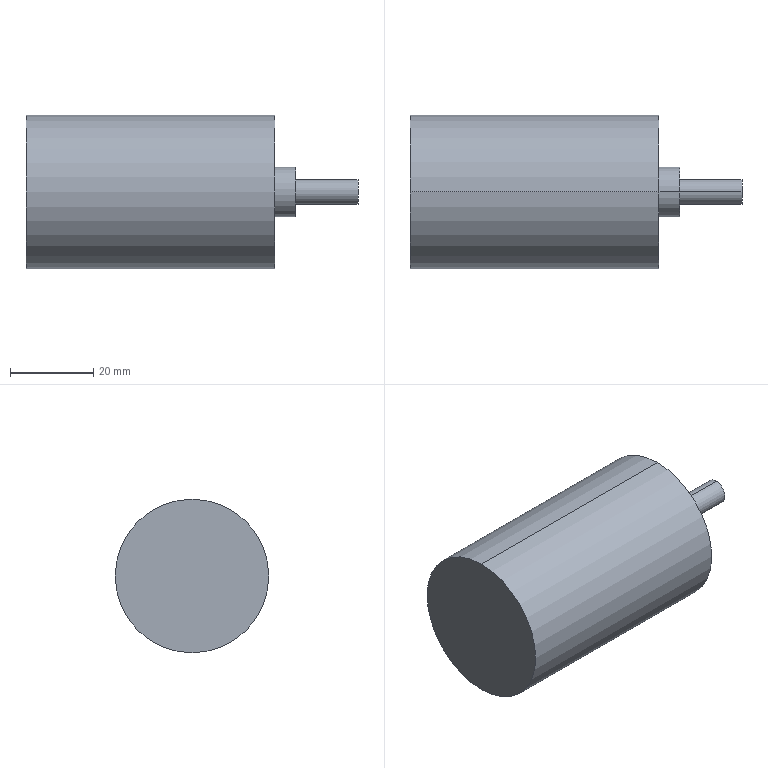Component | SolidWorks | AS-011-JG0105-1 | 1 solid | 34 faces | box 80 x 37 x 37 mm | volume 65244 mm3 | cylinder 18 | cone 12 | plane 4 | commonest cylinder face diameters 2.5 x12 6 x2 12 x2 37 x2
build123d program:
from build123d import *

# Parameters (mm, degrees)
M3_TAPPED_HOLE1_D     = 2.5
M3_TAPPED_HOLE1_DEPTH = 8.5
M3_TAPPED_HOLE1_TIP   = 0.7511


with BuildPart() as part:
    # Sketch1 → Revolve1 (revolve)
    with BuildSketch(Plane.XY, mode=Mode.PRIVATE) as revolve1_sk:
        Polygon((80, 3), (65, 3), (65, 6), (60, 6), (60, 18.5), (0, 18.5), (0, 0), (80, 0), align=None)
    revolve(revolve1_sk.sketch.rotate(Axis((80, 0, 0), (-1, 0, 0)), 90), axis=Axis((80, 0, 0), (-1, 0, 0)))

    # M3 Tapped Hole1
    with Locations(Plane(origin=(60, 0, 0), x_dir=(0, 0, -1), z_dir=(1, 0, 0))):
        with Locations((7.75, 13.423), (-7.75, 13.423), (15.5, 0), (-15.5, 0), (-7.75, -13.423), (7.75, -13.423)):
            Hole(M3_TAPPED_HOLE1_D / 2, depth=M3_TAPPED_HOLE1_DEPTH)
            with Locations((0, 0, -(M3_TAPPED_HOLE1_DEPTH + M3_TAPPED_HOLE1_TIP / 2))):  # 118° drill point
                Cone(0, M3_TAPPED_HOLE1_D / 2, M3_TAPPED_HOLE1_TIP, mode=Mode.SUBTRACT)


solid = part.part

# Placed as in the assembly
solid = solid.moved(Location((-97, -18, -10), (0, 0, 0)))
STEP:
#1=CARTESIAN_POINT('',(-1.791,-0.1802,-0.6496));
#2=VERTEX_POINT('',#1);
#3=CARTESIAN_POINT('',(-1.791,-0.1802,-0.748));
#4=VERTEX_POINT('',#3);
#5=CARTESIAN_POINT('',(-1.791,-0.1802,-0.6988));
#6=DIRECTION('',(1.,0.,0.));
#7=DIRECTION('',(0.,0.,-1.));
#8=AXIS2_PLACEMENT_3D('',#5,#6,#7);
#9=CIRCLE('',#8,0.04921);
#10=EDGE_CURVE('',#2,#4,#9,.T.);
#11=ORIENTED_EDGE('',*,*,#10,.F.);
#12=CARTESIAN_POINT('',(-1.457,-0.1802,-0.6496));
#13=VERTEX_POINT('',#12);
#14=CARTESIAN_POINT('',(-1.457,-0.1802,-0.6496));
#15=DIRECTION('',(1.,0.,0.));
#16=VECTOR('',#15,39.37);
#17=LINE('',#14,#16);
#18=EDGE_CURVE('',#2,#13,#17,.T.);
#19=ORIENTED_EDGE('',*,*,#18,.T.);
#20=CARTESIAN_POINT('',(-1.457,-0.1802,-0.748));
#21=VERTEX_POINT('',#20);
#22=CARTESIAN_POINT('',(-1.457,-0.1802,-0.6988));
#23=DIRECTION('',(1.,0.,0.));
#24=DIRECTION('',(0.,0.,-1.));
#25=AXIS2_PLACEMENT_3D('',#22,#23,#24);
#26=CIRCLE('',#25,0.04921);
#27=EDGE_CURVE('',#13,#21,#26,.T.);
#28=ORIENTED_EDGE('',*,*,#27,.T.);
#29=CARTESIAN_POINT('',(-1.457,-0.1802,-0.748));
#30=DIRECTION('',(1.,0.,0.));
#31=VECTOR('',#30,39.37);
#32=LINE('',#29,#31);
#33=EDGE_CURVE('',#4,#21,#32,.T.);
#34=ORIENTED_EDGE('',*,*,#33,.F.);
#35=EDGE_LOOP('',(#11,#19,#28,#34));
#36=FACE_OUTER_BOUND('',#35,.T.);
#37=CARTESIAN_POINT('',(-1.457,-0.1802,-0.6988));
#38=DIRECTION('',(1.,0.,0.));
#39=DIRECTION('',(0.,0.,-1.));
#40=AXIS2_PLACEMENT_3D('',#37,#38,#39);
#41=CYLINDRICAL_SURFACE('',#40,0.04921);
#42=ADVANCED_FACE('',(#36),#41,.F.);
#43=CARTESIAN_POINT('',(-1.821,-0.1802,-0.6988));
#44=VERTEX_POINT('',#43);
#45=CARTESIAN_POINT('',(-1.791,-0.1802,-0.748));
#46=DIRECTION('',(0.515,0.,-0.8572));
#47=VECTOR('',#46,39.37);
#48=LINE('',#45,#47);
#49=EDGE_CURVE('',#44,#4,#48,.T.);
#50=ORIENTED_EDGE('',*,*,#49,.F.);
#51=CARTESIAN_POINT('',(-1.791,-0.1802,-0.6496));
#52=DIRECTION('',(0.515,0.,0.8572));
#53=VECTOR('',#52,39.37);
#54=LINE('',#51,#53);
#55=EDGE_CURVE('',#44,#2,#54,.T.);
#56=ORIENTED_EDGE('',*,*,#55,.T.);
#57=ORIENTED_EDGE('',*,*,#10,.T.);
#58=EDGE_LOOP('',(#50,#56,#57));
#59=FACE_OUTER_BOUND('',#58,.T.);
#60=CARTESIAN_POINT('',(-1.791,-0.1802,-0.6988));
#61=DIRECTION('',(1.,0.,0.));
#62=DIRECTION('',(0.,0.,-1.));
#63=AXIS2_PLACEMENT_3D('',#60,#61,#62);
#64=CONICAL_SURFACE('',#63,0.04921,1.03);
#65=ADVANCED_FACE('',(#59),#64,.F.);
#66=CARTESIAN_POINT('',(-1.791,-0.1802,-0.03937));
#67=VERTEX_POINT('',#66);
#68=CARTESIAN_POINT('',(-1.791,-0.1802,-0.1378));
#69=VERTEX_POINT('',#68);
#70=CARTESIAN_POINT('',(-1.791,-0.1802,-0.08858));
#71=DIRECTION('',(1.,0.,0.));
#72=DIRECTION('',(0.,0.,-1.));
#73=AXIS2_PLACEMENT_3D('',#70,#71,#72);
#74=CIRCLE('',#73,0.04921);
#75=EDGE_CURVE('',#67,#69,#74,.T.);
#76=ORIENTED_EDGE('',*,*,#75,.F.);
#77=CARTESIAN_POINT('',(-1.457,-0.1802,-0.03937));
#78=VERTEX_POINT('',#77);
#79=CARTESIAN_POINT('',(-1.457,-0.1802,-0.03937));
#80=DIRECTION('',(1.,0.,0.));
#81=VECTOR('',#80,39.37);
#82=LINE('',#79,#81);
#83=EDGE_CURVE('',#67,#78,#82,.T.);
#84=ORIENTED_EDGE('',*,*,#83,.T.);
#85=CARTESIAN_POINT('',(-1.457,-0.1802,-0.1378));
#86=VERTEX_POINT('',#85);
#87=CARTESIAN_POINT('',(-1.457,-0.1802,-0.08858));
#88=DIRECTION('',(1.,0.,0.));
#89=DIRECTION('',(0.,0.,-1.));
#90=AXIS2_PLACEMENT_3D('',#87,#88,#89);
#91=CIRCLE('',#90,0.04921);
#92=EDGE_CURVE('',#78,#86,#91,.T.);
#93=ORIENTED_EDGE('',*,*,#92,.T.);
#94=CARTESIAN_POINT('',(-1.457,-0.1802,-0.1378));
#95=DIRECTION('',(1.,0.,0.));
#96=VECTOR('',#95,39.37);
#97=LINE('',#94,#96);
#98=EDGE_CURVE('',#69,#86,#97,.T.);
#99=ORIENTED_EDGE('',*,*,#98,.F.);
#100=EDGE_LOOP('',(#76,#84,#93,#99));
#101=FACE_OUTER_BOUND('',#100,.T.);
#102=CARTESIAN_POINT('',(-1.457,-0.1802,-0.08858));
#103=DIRECTION('',(1.,0.,0.));
#104=DIRECTION('',(0.,0.,-1.));
#105=AXIS2_PLACEMENT_3D('',#102,#103,#104);
#106=CYLINDRICAL_SURFACE('',#105,0.04921);
#107=ADVANCED_FACE('',(#101),#106,.F.);
#108=CARTESIAN_POINT('',(-1.821,-0.1802,-0.08858));
#109=VERTEX_POINT('',#108);
#110=CARTESIAN_POINT('',(-1.791,-0.1802,-0.1378));
#111=DIRECTION('',(0.515,0.,-0.8572));
#112=VECTOR('',#111,39.37);
#113=LINE('',#110,#112);
#114=EDGE_CURVE('',#109,#69,#113,.T.);
#115=ORIENTED_EDGE('',*,*,#114,.F.);
#116=CARTESIAN_POINT('',(-1.791,-0.1802,-0.03937));
#117=DIRECTION('',(0.515,0.,0.8572));
#118=VECTOR('',#117,39.37);
#119=LINE('',#116,#118);
#120=EDGE_CURVE('',#109,#67,#119,.T.);
#121=ORIENTED_EDGE('',*,*,#120,.T.);
#122=ORIENTED_EDGE('',*,*,#75,.T.);
#123=EDGE_LOOP('',(#115,#121,#122));
#124=FACE_OUTER_BOUND('',#123,.T.);
#125=CARTESIAN_POINT('',(-1.791,-0.1802,-0.08858));
#126=DIRECTION('',(1.,0.,0.));
#127=DIRECTION('',(0.,0.,-1.));
#128=AXIS2_PLACEMENT_3D('',#125,#126,#127);
#129=CONICAL_SURFACE('',#128,0.04921,1.03);
#130=ADVANCED_FACE('',(#124),#129,.F.);
#131=CARTESIAN_POINT('',(-1.791,-0.7087,-0.9547));
#132=VERTEX_POINT('',#131);
#133=CARTESIAN_POINT('',(-1.791,-0.7087,-1.053));
#134=VERTEX_POINT('',#133);
#135=CARTESIAN_POINT('',(-1.791,-0.7087,-1.004));
#136=DIRECTION('',(1.,0.,0.));
#137=DIRECTION('',(0.,0.,-1.));
#138=AXIS2_PLACEMENT_3D('',#135,#136,#137);
#139=CIRCLE('',#138,0.04921);
#140=EDGE_CURVE('',#132,#134,#139,.T.);
#141=ORIENTED_EDGE('',*,*,#140,.F.);
#142=CARTESIAN_POINT('',(-1.457,-0.7087,-0.9547));
#143=VERTEX_POINT('',#142);
#144=CARTESIAN_POINT('',(-1.457,-0.7087,-0.9547));
#145=DIRECTION('',(1.,0.,0.));
#146=VECTOR('',#145,39.37);
#147=LINE('',#144,#146);
#148=EDGE_CURVE('',#132,#143,#147,.T.);
#149=ORIENTED_EDGE('',*,*,#148,.T.);
#150=CARTESIAN_POINT('',(-1.457,-0.7087,-1.053));
#151=VERTEX_POINT('',#150);
#152=CARTESIAN_POINT('',(-1.457,-0.7087,-1.004));
#153=DIRECTION('',(1.,0.,0.));
#154=DIRECTION('',(0.,0.,-1.));
#155=AXIS2_PLACEMENT_3D('',#152,#153,#154);
#156=CIRCLE('',#155,0.04921);
#157=EDGE_CURVE('',#143,#151,#156,.T.);
#158=ORIENTED_EDGE('',*,*,#157,.T.);
#159=CARTESIAN_POINT('',(-1.457,-0.7087,-1.053));
#160=DIRECTION('',(1.,0.,0.));
#161=VECTOR('',#160,39.37);
#162=LINE('',#159,#161);
#163=EDGE_CURVE('',#134,#151,#162,.T.);
#164=ORIENTED_EDGE('',*,*,#163,.F.);
#165=EDGE_LOOP('',(#141,#149,#158,#164));
#166=FACE_OUTER_BOUND('',#165,.T.);
#167=CARTESIAN_POINT('',(-1.457,-0.7087,-1.004));
#168=DIRECTION('',(1.,0.,0.));
#169=DIRECTION('',(0.,0.,-1.));
#170=AXIS2_PLACEMENT_3D('',#167,#168,#169);
#171=CYLINDRICAL_SURFACE('',#170,0.04921);
#172=ADVANCED_FACE('',(#166),#171,.F.);
#173=CARTESIAN_POINT('',(-1.821,-0.7087,-1.004));
#174=VERTEX_POINT('',#173);
#175=CARTESIAN_POINT('',(-1.791,-0.7087,-1.053));
#176=DIRECTION('',(0.515,0.,-0.8572));
#177=VECTOR('',#176,39.37);
#178=LINE('',#175,#177);
#179=EDGE_CURVE('',#174,#134,#178,.T.);
#180=ORIENTED_EDGE('',*,*,#179,.F.);
#181=CARTESIAN_POINT('',(-1.791,-0.7087,-0.9547));
#182=DIRECTION('',(0.515,0.,0.8572));
#183=VECTOR('',#182,39.37);
#184=LINE('',#181,#183);
#185=EDGE_CURVE('',#174,#132,#184,.T.);
#186=ORIENTED_EDGE('',*,*,#185,.T.);
#187=ORIENTED_EDGE('',*,*,#140,.T.);
#188=EDGE_LOOP('',(#180,#186,#187));
#189=FACE_OUTER_BOUND('',#188,.T.);
#190=CARTESIAN_POINT('',(-1.791,-0.7087,-1.004));
#191=DIRECTION('',(1.,0.,0.));
#192=DIRECTION('',(0.,0.,-1.));
#193=AXIS2_PLACEMENT_3D('',#190,#191,#192);
#194=CONICAL_SURFACE('',#193,0.04921,1.03);
#195=ADVANCED_FACE('',(#189),#194,.F.);
#196=CARTESIAN_POINT('',(-1.791,-0.7087,0.2657));
#197=VERTEX_POINT('',#196);
#198=CARTESIAN_POINT('',(-1.791,-0.7087,0.1673));
#199=VERTEX_POINT('',#198);
#200=CARTESIAN_POINT('',(-1.791,-0.7087,0.2165));
#201=DIRECTION('',(1.,0.,0.));
#202=DIRECTION('',(0.,0.,-1.));
#203=AXIS2_PLACEMENT_3D('',#200,#201,#202);
#204=CIRCLE('',#203,0.04921);
#205=EDGE_CURVE('',#197,#199,#204,.T.);
#206=ORIENTED_EDGE('',*,*,#205,.F.);
#207=CARTESIAN_POINT('',(-1.457,-0.7087,0.2657));
#208=VERTEX_POINT('',#207);
#209=CARTESIAN_POINT('',(-1.457,-0.7087,0.2657));
#210=DIRECTION('',(1.,0.,0.));
#211=VECTOR('',#210,39.37);
#212=LINE('',#209,#211);
#213=EDGE_CURVE('',#197,#208,#212,.T.);
#214=ORIENTED_EDGE('',*,*,#213,.T.);
#215=CARTESIAN_POINT('',(-1.457,-0.7087,0.1673));
#216=VERTEX_POINT('',#215);
#217=CARTESIAN_POINT('',(-1.457,-0.7087,0.2165));
#218=DIRECTION('',(1.,0.,0.));
#219=DIRECTION('',(0.,0.,-1.));
#220=AXIS2_PLACEMENT_3D('',#217,#218,#219);
#221=CIRCLE('',#220,0.04921);
#222=EDGE_CURVE('',#208,#216,#221,.T.);
#223=ORIENTED_EDGE('',*,*,#222,.T.);
#224=CARTESIAN_POINT('',(-1.457,-0.7087,0.1673));
#225=DIRECTION('',(1.,0.,0.));
#226=VECTOR('',#225,39.37);
#227=LINE('',#224,#226);
#228=EDGE_CURVE('',#199,#216,#227,.T.);
#229=ORIENTED_EDGE('',*,*,#228,.F.);
#230=EDGE_LOOP('',(#206,#214,#223,#229));
#231=FACE_OUTER_BOUND('',#230,.T.);
#232=CARTESIAN_POINT('',(-1.457,-0.7087,0.2165));
#233=DIRECTION('',(1.,0.,0.));
#234=DIRECTION('',(0.,0.,-1.));
#235=AXIS2_PLACEMENT_3D('',#232,#233,#234);
#236=CYLINDRICAL_SURFACE('',#235,0.04921);
#237=ADVANCED_FACE('',(#231),#236,.F.);
#238=CARTESIAN_POINT('',(-1.821,-0.7087,0.2165));
#239=VERTEX_POINT('',#238);
#240=CARTESIAN_POINT('',(-1.791,-0.7087,0.1673));
#241=DIRECTION('',(0.515,0.,-0.8572));
#242=VECTOR('',#241,39.37);
#243=LINE('',#240,#242);
#244=EDGE_CURVE('',#239,#199,#243,.T.);
#245=ORIENTED_EDGE('',*,*,#244,.F.);
#246=CARTESIAN_POINT('',(-1.791,-0.7087,0.2657));
#247=DIRECTION('',(0.515,0.,0.8572));
#248=VECTOR('',#247,39.37);
#249=LINE('',#246,#248);
#250=EDGE_CURVE('',#239,#197,#249,.T.);
#251=ORIENTED_EDGE('',*,*,#250,.T.);
#252=ORIENTED_EDGE('',*,*,#205,.T.);
#253=EDGE_LOOP('',(#245,#251,#252));
#254=FACE_OUTER_BOUND('',#253,.T.);
#255=CARTESIAN_POINT('',(-1.791,-0.7087,0.2165));
#256=DIRECTION('',(1.,0.,0.));
#257=DIRECTION('',(0.,0.,-1.));
#258=AXIS2_PLACEMENT_3D('',#255,#256,#257);
#259=CONICAL_SURFACE('',#258,0.04921,1.03);
#260=ADVANCED_FACE('',(#254),#259,.F.);
#261=CARTESIAN_POINT('',(-1.791,-1.237,-0.03937));
#262=VERTEX_POINT('',#261);
#263=CARTESIAN_POINT('',(-1.791,-1.237,-0.1378));
#264=VERTEX_POINT('',#263);
#265=CARTESIAN_POINT('',(-1.791,-1.237,-0.08858));
#266=DIRECTION('',(1.,0.,0.));
#267=DIRECTION('',(0.,0.,-1.));
#268=AXIS2_PLACEMENT_3D('',#265,#266,#267);
#269=CIRCLE('',#268,0.04921);
#270=EDGE_CURVE('',#262,#264,#269,.T.);
#271=ORIENTED_EDGE('',*,*,#270,.F.);
#272=CARTESIAN_POINT('',(-1.457,-1.237,-0.03937));
#273=VERTEX_POINT('',#272);
#274=CARTESIAN_POINT('',(-1.457,-1.237,-0.03937));
#275=DIRECTION('',(1.,0.,0.));
#276=VECTOR('',#275,39.37);
#277=LINE('',#274,#276);
#278=EDGE_CURVE('',#262,#273,#277,.T.);
#279=ORIENTED_EDGE('',*,*,#278,.T.);
#280=CARTESIAN_POINT('',(-1.457,-1.237,-0.1378));
#281=VERTEX_POINT('',#280);
#282=CARTESIAN_POINT('',(-1.457,-1.237,-0.08858));
#283=DIRECTION('',(1.,0.,0.));
#284=DIRECTION('',(0.,0.,-1.));
#285=AXIS2_PLACEMENT_3D('',#282,#283,#284);
#286=CIRCLE('',#285,0.04921);
#287=EDGE_CURVE('',#273,#281,#286,.T.);
#288=ORIENTED_EDGE('',*,*,#287,.T.);
#289=CARTESIAN_POINT('',(-1.457,-1.237,-0.1378));
#290=DIRECTION('',(1.,0.,0.));
#291=VECTOR('',#290,39.37);
#292=LINE('',#289,#291);
#293=EDGE_CURVE('',#264,#281,#292,.T.);
#294=ORIENTED_EDGE('',*,*,#293,.F.);
#295=EDGE_LOOP('',(#271,#279,#288,#294));
#296=FACE_OUTER_BOUND('',#295,.T.);
#297=CARTESIAN_POINT('',(-1.457,-1.237,-0.08858));
#298=DIRECTION('',(1.,0.,0.));
#299=DIRECTION('',(0.,0.,-1.));
#300=AXIS2_PLACEMENT_3D('',#297,#298,#299);
#301=CYLINDRICAL_SURFACE('',#300,0.04921);
#302=ADVANCED_FACE('',(#296),#301,.F.);
#303=CARTESIAN_POINT('',(-1.821,-1.237,-0.08858));
#304=VERTEX_POINT('',#303);
#305=CARTESIAN_POINT('',(-1.791,-1.237,-0.1378));
#306=DIRECTION('',(0.515,0.,-0.8572));
#307=VECTOR('',#306,39.37);
#308=LINE('',#305,#307);
#309=EDGE_CURVE('',#304,#264,#308,.T.);
#310=ORIENTED_EDGE('',*,*,#309,.F.);
#311=CARTESIAN_POINT('',(-1.791,-1.237,-0.03937));
#312=DIRECTION('',(0.515,0.,0.8572));
#313=VECTOR('',#312,39.37);
#314=LINE('',#311,#313);
#315=EDGE_CURVE('',#304,#262,#314,.T.);
#316=ORIENTED_EDGE('',*,*,#315,.T.);
#317=ORIENTED_EDGE('',*,*,#270,.T.);
#318=EDGE_LOOP('',(#310,#316,#317));
#319=FACE_OUTER_BOUND('',#318,.T.);
#320=CARTESIAN_POINT('',(-1.791,-1.237,-0.08858));
#321=DIRECTION('',(1.,0.,0.));
#322=DIRECTION('',(0.,0.,-1.));
#323=AXIS2_PLACEMENT_3D('',#320,#321,#322);
#324=CONICAL_SURFACE('',#323,0.04921,1.03);
#325=ADVANCED_FACE('',(#319),#324,.F.);
#326=CARTESIAN_POINT('',(-1.791,-1.237,-0.6496));
#327=VERTEX_POINT('',#326);
#328=CARTESIAN_POINT('',(-1.791,-1.237,-0.748));
#329=VERTEX_POINT('',#328);
#330=CARTESIAN_POINT('',(-1.791,-1.237,-0.6988));
#331=DIRECTION('',(1.,0.,0.));
#332=DIRECTION('',(0.,0.,-1.));
#333=AXIS2_PLACEMENT_3D('',#330,#331,#332);
#334=CIRCLE('',#333,0.04921);
#335=EDGE_CURVE('',#327,#329,#334,.T.);
#336=ORIENTED_EDGE('',*,*,#335,.F.);
#337=CARTESIAN_POINT('',(-1.457,-1.237,-0.6496));
#338=VERTEX_POINT('',#337);
#339=CARTESIAN_POINT('',(-1.457,-1.237,-0.6496));
#340=DIRECTION('',(1.,0.,0.));
#341=VECTOR('',#340,39.37);
#342=LINE('',#339,#341);
#343=EDGE_CURVE('',#327,#338,#342,.T.);
#344=ORIENTED_EDGE('',*,*,#343,.T.);
#345=CARTESIAN_POINT('',(-1.457,-1.237,-0.748));
#346=VERTEX_POINT('',#345);
#347=CARTESIAN_POINT('',(-1.457,-1.237,-0.6988));
#348=DIRECTION('',(1.,0.,0.));
#349=DIRECTION('',(0.,0.,-1.));
#350=AXIS2_PLACEMENT_3D('',#347,#348,#349);
#351=CIRCLE('',#350,0.04921);
#352=EDGE_CURVE('',#338,#346,#351,.T.);
#353=ORIENTED_EDGE('',*,*,#352,.T.);
#354=CARTESIAN_POINT('',(-1.457,-1.237,-0.748));
#355=DIRECTION('',(1.,0.,0.));
#356=VECTOR('',#355,39.37);
#357=LINE('',#354,#356);
#358=EDGE_CURVE('',#329,#346,#357,.T.);
#359=ORIENTED_EDGE('',*,*,#358,.F.);
#360=EDGE_LOOP('',(#336,#344,#353,#359));
#361=FACE_OUTER_BOUND('',#360,.T.);
#362=CARTESIAN_POINT('',(-1.457,-1.237,-0.6988));
#363=DIRECTION('',(1.,0.,0.));
#364=DIRECTION('',(0.,0.,-1.));
#365=AXIS2_PLACEMENT_3D('',#362,#363,#364);
#366=CYLINDRICAL_SURFACE('',#365,0.04921);
#367=ADVANCED_FACE('',(#361),#366,.F.);
#368=CARTESIAN_POINT('',(-1.821,-1.237,-0.6988));
#369=VERTEX_POINT('',#368);
#370=CARTESIAN_POINT('',(-1.791,-1.237,-0.748));
#371=DIRECTION('',(0.515,0.,-0.8572));
#372=VECTOR('',#371,39.37);
#373=LINE('',#370,#372);
#374=EDGE_CURVE('',#369,#329,#373,.T.);
#375=ORIENTED_EDGE('',*,*,#374,.F.);
#376=CARTESIAN_POINT('',(-1.791,-1.237,-0.6496));
#377=DIRECTION('',(0.515,0.,0.8572));
#378=VECTOR('',#377,39.37);
#379=LINE('',#376,#378);
#380=EDGE_CURVE('',#369,#327,#379,.T.);
#381=ORIENTED_EDGE('',*,*,#380,.T.);
#382=ORIENTED_EDGE('',*,*,#335,.T.);
#383=EDGE_LOOP('',(#375,#381,#382));
#384=FACE_OUTER_BOUND('',#383,.T.);
#385=CARTESIAN_POINT('',(-1.791,-1.237,-0.6988));
#386=DIRECTION('',(1.,0.,0.));
#387=DIRECTION('',(0.,0.,-1.));
#388=AXIS2_PLACEMENT_3D('',#385,#386,#387);
#389=CONICAL_SURFACE('',#388,0.04921,1.03);
#390=ADVANCED_FACE('',(#384),#389,.F.);
#391=CARTESIAN_POINT('',(-1.26,-0.7087,-0.5118));
#392=VERTEX_POINT('',#391);
#393=CARTESIAN_POINT('',(-1.26,-0.7087,-0.2756));
#394=VERTEX_POINT('',#393);
#395=CARTESIAN_POINT('',(-1.26,-0.7087,-0.3937));
#396=DIRECTION('',(1.,0.,0.));
#397=DIRECTION('',(0.,0.,-1.));
#398=AXIS2_PLACEMENT_3D('',#395,#396,#397);
#399=CIRCLE('',#398,0.1181);
#400=EDGE_CURVE('',#392,#394,#399,.T.);
#401=ORIENTED_EDGE('',*,*,#400,.T.);
#402=CARTESIAN_POINT('',(-0.6693,-0.7087,-0.2756));
#403=VERTEX_POINT('',#402);
#404=CARTESIAN_POINT('',(-0.6693,-0.7087,-0.2756));
#405=DIRECTION('',(1.,0.,0.));
#406=VECTOR('',#405,39.37);
#407=LINE('',#404,#406);
#408=EDGE_CURVE('',#394,#403,#407,.T.);
#409=ORIENTED_EDGE('',*,*,#408,.T.);
#410=CARTESIAN_POINT('',(-0.6693,-0.7087,-0.5118));
#411=VERTEX_POINT('',#410);
#412=CARTESIAN_POINT('',(-0.6693,-0.7087,-0.3937));
#413=DIRECTION('',(1.,0.,0.));
#414=DIRECTION('',(0.,0.,-1.));
#415=AXIS2_PLACEMENT_3D('',#412,#413,#414);
#416=CIRCLE('',#415,0.1181);
#417=EDGE_CURVE('',#411,#403,#416,.T.);
#418=ORIENTED_EDGE('',*,*,#417,.F.);
#419=CARTESIAN_POINT('',(-0.6693,-0.7087,-0.5118));
#420=DIRECTION('',(1.,0.,0.));
#421=VECTOR('',#420,39.37);
#422=LINE('',#419,#421);
#423=EDGE_CURVE('',#392,#411,#422,.T.);
#424=ORIENTED_EDGE('',*,*,#423,.F.);
#425=EDGE_LOOP('',(#401,#409,#418,#424));
#426=FACE_OUTER_BOUND('',#425,.T.);
#427=CARTESIAN_POINT('',(-0.6693,-0.7087,-0.3937));
#428=DIRECTION('',(1.,0.,0.));
#429=DIRECTION('',(0.,0.,-1.));
#430=AXIS2_PLACEMENT_3D('',#427,#428,#429);
#431=CYLINDRICAL_SURFACE('',#430,0.1181);
#432=ADVANCED_FACE('',(#426),#431,.T.);
#433=CARTESIAN_POINT('',(-1.457,-0.7087,-0.6299));
#434=VERTEX_POINT('',#433);
#435=CARTESIAN_POINT('',(-1.457,-0.7087,-0.1575));
#436=VERTEX_POINT('',#435);
#437=CARTESIAN_POINT('',(-1.457,-0.7087,-0.3937));
#438=DIRECTION('',(1.,0.,0.));
#439=DIRECTION('',(0.,0.,-1.));
#440=AXIS2_PLACEMENT_3D('',#437,#438,#439);
#441=CIRCLE('',#440,0.2362);
#442=EDGE_CURVE('',#434,#436,#441,.T.);
#443=ORIENTED_EDGE('',*,*,#442,.T.);
#444=CARTESIAN_POINT('',(-1.26,-0.7087,-0.1575));
#445=VERTEX_POINT('',#444);
#446=CARTESIAN_POINT('',(-0.6693,-0.7087,-0.1575));
#447=DIRECTION('',(1.,0.,0.));
#448=VECTOR('',#447,39.37);
#449=LINE('',#446,#448);
#450=EDGE_CURVE('',#436,#445,#449,.T.);
#451=ORIENTED_EDGE('',*,*,#450,.T.);
#452=CARTESIAN_POINT('',(-1.26,-0.7087,-0.6299));
#453=VERTEX_POINT('',#452);
#454=CARTESIAN_POINT('',(-1.26,-0.7087,-0.3937));
#455=DIRECTION('',(1.,0.,0.));
#456=DIRECTION('',(0.,0.,-1.));
#457=AXIS2_PLACEMENT_3D('',#454,#455,#456);
#458=CIRCLE('',#457,0.2362);
#459=EDGE_CURVE('',#453,#445,#458,.T.);
#460=ORIENTED_EDGE('',*,*,#459,.F.);
#461=CARTESIAN_POINT('',(-0.6693,-0.7087,-0.6299));
#462=DIRECTION('',(1.,0.,0.));
#463=VECTOR('',#462,39.37);
#464=LINE('',#461,#463);
#465=EDGE_CURVE('',#434,#453,#464,.T.);
#466=ORIENTED_EDGE('',*,*,#465,.F.);
#467=EDGE_LOOP('',(#443,#451,#460,#466));
#468=FACE_OUTER_BOUND('',#467,.T.);
#469=CARTESIAN_POINT('',(-0.6693,-0.7087,-0.3937));
#470=DIRECTION('',(1.,0.,0.));
#471=DIRECTION('',(0.,0.,-1.));
#472=AXIS2_PLACEMENT_3D('',#469,#470,#471);
#473=CYLINDRICAL_SURFACE('',#472,0.2362);
#474=ADVANCED_FACE('',(#468),#473,.T.);
#475=CARTESIAN_POINT('',(-3.819,-0.7087,-1.122));
#476=VERTEX_POINT('',#475);
#477=CARTESIAN_POINT('',(-3.819,-0.7087,0.3346));
#478=VERTEX_POINT('',#477);
#479=CARTESIAN_POINT('',(-3.819,-0.7087,-0.3937));
#480=DIRECTION('',(1.,0.,0.));
#481=DIRECTION('',(0.,0.,-1.));
#482=AXIS2_PLACEMENT_3D('',#479,#480,#481);
#483=CIRCLE('',#482,0.7283);
#484=EDGE_CURVE('',#476,#478,#483,.T.);
#485=ORIENTED_EDGE('',*,*,#484,.T.);
#486=CARTESIAN_POINT('',(-1.457,-0.7087,0.3346));
#487=VERTEX_POINT('',#486);
#488=CARTESIAN_POINT('',(-0.6693,-0.7087,0.3346));
#489=DIRECTION('',(1.,0.,0.));
#490=VECTOR('',#489,39.37);
#491=LINE('',#488,#490);
#492=EDGE_CURVE('',#478,#487,#491,.T.);
#493=ORIENTED_EDGE('',*,*,#492,.T.);
#494=CARTESIAN_POINT('',(-1.457,-0.7087,-1.122));
#495=VERTEX_POINT('',#494);
#496=CARTESIAN_POINT('',(-1.457,-0.7087,-0.3937));
#497=DIRECTION('',(1.,0.,0.));
#498=DIRECTION('',(0.,0.,-1.));
#499=AXIS2_PLACEMENT_3D('',#496,#497,#498);
#500=CIRCLE('',#499,0.7283);
#501=EDGE_CURVE('',#495,#487,#500,.T.);
#502=ORIENTED_EDGE('',*,*,#501,.F.);
#503=CARTESIAN_POINT('',(-0.6693,-0.7087,-1.122));
#504=DIRECTION('',(1.,0.,0.));
#505=VECTOR('',#504,39.37);
#506=LINE('',#503,#505);
#507=EDGE_CURVE('',#476,#495,#506,.T.);
#508=ORIENTED_EDGE('',*,*,#507,.F.);
#509=EDGE_LOOP('',(#485,#493,#502,#508));
#510=FACE_OUTER_BOUND('',#509,.T.);
#511=CARTESIAN_POINT('',(-0.6693,-0.7087,-0.3937));
#512=DIRECTION('',(1.,0.,0.));
#513=DIRECTION('',(0.,0.,-1.));
#514=AXIS2_PLACEMENT_3D('',#511,#512,#513);
#515=CYLINDRICAL_SURFACE('',#514,0.7283);
#516=ADVANCED_FACE('',(#510),#515,.T.);
#517=ORIENTED_EDGE('',*,*,#417,.T.);
#518=CARTESIAN_POINT('',(-0.6693,-0.7087,-0.3937));
#519=DIRECTION('',(1.,0.,0.));
#520=DIRECTION('',(0.,0.,-1.));
#521=AXIS2_PLACEMENT_3D('',#518,#519,#520);
#522=CIRCLE('',#521,0.1181);
#523=EDGE_CURVE('',#403,#411,#522,.T.);
#524=ORIENTED_EDGE('',*,*,#523,.T.);
#525=EDGE_LOOP('',(#517,#524));
#526=FACE_OUTER_BOUND('',#525,.T.);
#527=CARTESIAN_POINT('',(-0.6693,-0.5906,-0.3937));
#528=DIRECTION('',(1.,0.,0.));
#529=DIRECTION('',(0.,0.,-1.));
#530=AXIS2_PLACEMENT_3D('',#527,#528,#529);
#531=PLANE('',#530);
#532=ADVANCED_FACE('',(#526),#531,.T.);
#533=ORIENTED_EDGE('',*,*,#484,.F.);
#534=CARTESIAN_POINT('',(-3.819,-0.7087,-0.3937));
#535=DIRECTION('',(1.,0.,0.));
#536=DIRECTION('',(0.,0.,-1.));
#537=AXIS2_PLACEMENT_3D('',#534,#535,#536);
#538=CIRCLE('',#537,0.7283);
#539=EDGE_CURVE('',#478,#476,#538,.T.);
#540=ORIENTED_EDGE('',*,*,#539,.F.);
#541=EDGE_LOOP('',(#533,#540));
#542=FACE_OUTER_BOUND('',#541,.T.);
#543=CARTESIAN_POINT('',(-3.819,0.01969,-0.3937));
#544=DIRECTION('',(-1.,0.,0.));
#545=DIRECTION('',(0.,0.,1.));
#546=AXIS2_PLACEMENT_3D('',#543,#544,#545);
#547=PLANE('',#546);
#548=ADVANCED_FACE('',(#542),#547,.T.);
#549=ORIENTED_EDGE('',*,*,#492,.F.);
#550=ORIENTED_EDGE('',*,*,#539,.T.);
#551=ORIENTED_EDGE('',*,*,#507,.T.);
#552=CARTESIAN_POINT('',(-1.457,-0.7087,-0.3937));
#553=DIRECTION('',(1.,0.,0.));
#554=DIRECTION('',(0.,0.,-1.));
#555=AXIS2_PLACEMENT_3D('',#552,#553,#554);
#556=CIRCLE('',#555,0.7283);
#557=EDGE_CURVE('',#487,#495,#556,.T.);
#558=ORIENTED_EDGE('',*,*,#557,.F.);
#559=EDGE_LOOP('',(#549,#550,#551,#558));
#560=FACE_OUTER_BOUND('',#559,.T.);
#561=CARTESIAN_POINT('',(-0.6693,-0.7087,-0.3937));
#562=DIRECTION('',(1.,0.,0.));
#563=DIRECTION('',(0.,0.,-1.));
#564=AXIS2_PLACEMENT_3D('',#561,#562,#563);
#565=CYLINDRICAL_SURFACE('',#564,0.7283);
#566=ADVANCED_FACE('',(#560),#565,.T.);
#567=CARTESIAN_POINT('',(-1.457,-0.1802,-0.6988));
#568=DIRECTION('',(1.,0.,0.));
#569=DIRECTION('',(0.,0.,-1.));
#570=AXIS2_PLACEMENT_3D('',#567,#568,#569);
#571=CIRCLE('',#570,0.04921);
#572=EDGE_CURVE('',#21,#13,#571,.T.);
#573=ORIENTED_EDGE('',*,*,#572,.F.);
#574=ORIENTED_EDGE('',*,*,#27,.F.);
#575=EDGE_LOOP('',(#573,#574));
#576=FACE_BOUND('',#575,.T.);
#577=CARTESIAN_POINT('',(-1.457,-0.1802,-0.08858));
#578=DIRECTION('',(1.,0.,0.));
#579=DIRECTION('',(0.,0.,-1.));
#580=AXIS2_PLACEMENT_3D('',#577,#578,#579);
#581=CIRCLE('',#580,0.04921);
#582=EDGE_CURVE('',#86,#78,#581,.T.);
#583=ORIENTED_EDGE('',*,*,#582,.F.);
#584=ORIENTED_EDGE('',*,*,#92,.F.);
#585=EDGE_LOOP('',(#583,#584));
#586=FACE_BOUND('',#585,.T.);
#587=CARTESIAN_POINT('',(-1.457,-0.7087,-1.004));
#588=DIRECTION('',(1.,0.,0.));
#589=DIRECTION('',(0.,0.,-1.));
#590=AXIS2_PLACEMENT_3D('',#587,#588,#589);
#591=CIRCLE('',#590,0.04921);
#592=EDGE_CURVE('',#151,#143,#591,.T.);
#593=ORIENTED_EDGE('',*,*,#592,.F.);
#594=ORIENTED_EDGE('',*,*,#157,.F.);
#595=EDGE_LOOP('',(#593,#594));
#596=FACE_BOUND('',#595,.T.);
#597=CARTESIAN_POINT('',(-1.457,-0.7087,0.2165));
#598=DIRECTION('',(1.,0.,0.));
#599=DIRECTION('',(0.,0.,-1.));
#600=AXIS2_PLACEMENT_3D('',#597,#598,#599);
#601=CIRCLE('',#600,0.04921);
#602=EDGE_CURVE('',#216,#208,#601,.T.);
#603=ORIENTED_EDGE('',*,*,#602,.F.);
#604=ORIENTED_EDGE('',*,*,#222,.F.);
#605=EDGE_LOOP('',(#603,#604));
#606=FACE_BOUND('',#605,.T.);
#607=CARTESIAN_POINT('',(-1.457,-1.237,-0.08858));
#608=DIRECTION('',(1.,0.,0.));
#609=DIRECTION('',(0.,0.,-1.));
#610=AXIS2_PLACEMENT_3D('',#607,#608,#609);
#611=CIRCLE('',#610,0.04921);
#612=EDGE_CURVE('',#281,#273,#611,.T.);
#613=ORIENTED_EDGE('',*,*,#612,.F.);
#614=ORIENTED_EDGE('',*,*,#287,.F.);
#615=EDGE_LOOP('',(#613,#614));
#616=FACE_BOUND('',#615,.T.);
#617=CARTESIAN_POINT('',(-1.457,-1.237,-0.6988));
#618=DIRECTION('',(1.,0.,0.));
#619=DIRECTION('',(0.,0.,-1.));
#620=AXIS2_PLACEMENT_3D('',#617,#618,#619);
#621=CIRCLE('',#620,0.04921);
#622=EDGE_CURVE('',#346,#338,#621,.T.);
#623=ORIENTED_EDGE('',*,*,#622,.F.);
#624=ORIENTED_EDGE('',*,*,#352,.F.);
#625=EDGE_LOOP('',(#623,#624));
#626=FACE_BOUND('',#625,.T.);
#627=ORIENTED_EDGE('',*,*,#501,.T.);
#628=ORIENTED_EDGE('',*,*,#557,.T.);
#629=EDGE_LOOP('',(#627,#628));
#630=FACE_OUTER_BOUND('',#629,.T.);
#631=ORIENTED_EDGE('',*,*,#442,.F.);
#632=CARTESIAN_POINT('',(-1.457,-0.7087,-0.3937));
#633=DIRECTION('',(1.,0.,0.));
#634=DIRECTION('',(0.,0.,-1.));
#635=AXIS2_PLACEMENT_3D('',#632,#633,#634);
#636=CIRCLE('',#635,0.2362);
#637=EDGE_CURVE('',#436,#434,#636,.T.);
#638=ORIENTED_EDGE('',*,*,#637,.F.);
#639=EDGE_LOOP('',(#631,#638));
#640=FACE_BOUND('',#639,.T.);
#641=CARTESIAN_POINT('',(-1.457,0.01969,-0.3937));
#642=DIRECTION('',(1.,0.,0.));
#643=DIRECTION('',(0.,0.,-1.));
#644=AXIS2_PLACEMENT_3D('',#641,#642,#643);
#645=PLANE('',#644);
#646=ADVANCED_FACE('',(#576,#586,#596,#606,#616,#626,#630,#640),#645,.T.);
#647=ORIENTED_EDGE('',*,*,#450,.F.);
#648=ORIENTED_EDGE('',*,*,#637,.T.);
#649=ORIENTED_EDGE('',*,*,#465,.T.);
#650=CARTESIAN_POINT('',(-1.26,-0.7087,-0.3937));
#651=DIRECTION('',(1.,0.,0.));
#652=DIRECTION('',(0.,0.,-1.));
#653=AXIS2_PLACEMENT_3D('',#650,#651,#652);
#654=CIRCLE('',#653,0.2362);
#655=EDGE_CURVE('',#445,#453,#654,.T.);
#656=ORIENTED_EDGE('',*,*,#655,.F.);
#657=EDGE_LOOP('',(#647,#648,#649,#656));
#658=FACE_OUTER_BOUND('',#657,.T.);
#659=CARTESIAN_POINT('',(-0.6693,-0.7087,-0.3937));
#660=DIRECTION('',(1.,0.,0.));
#661=DIRECTION('',(0.,0.,-1.));
#662=AXIS2_PLACEMENT_3D('',#659,#660,#661);
#663=CYLINDRICAL_SURFACE('',#662,0.2362);
#664=ADVANCED_FACE('',(#658),#663,.T.);
#665=ORIENTED_EDGE('',*,*,#459,.T.);
#666=ORIENTED_EDGE('',*,*,#655,.T.);
#667=EDGE_LOOP('',(#665,#666));
#668=FACE_OUTER_BOUND('',#667,.T.);
#669=ORIENTED_EDGE('',*,*,#400,.F.);
#670=CARTESIAN_POINT('',(-1.26,-0.7087,-0.3937));
#671=DIRECTION('',(1.,0.,0.));
#672=DIRECTION('',(0.,0.,-1.));
#673=AXIS2_PLACEMENT_3D('',#670,#671,#672);
#674=CIRCLE('',#673,0.1181);
#675=EDGE_CURVE('',#394,#392,#674,.T.);
#676=ORIENTED_EDGE('',*,*,#675,.F.);
#677=EDGE_LOOP('',(#669,#676));
#678=FACE_BOUND('',#677,.T.);
#679=CARTESIAN_POINT('',(-1.26,-0.4724,-0.3937));
#680=DIRECTION('',(1.,0.,0.));
#681=DIRECTION('',(0.,0.,-1.));
#682=AXIS2_PLACEMENT_3D('',#679,#680,#681);
#683=PLANE('',#682);
#684=ADVANCED_FACE('',(#668,#678),#683,.T.);
#685=ORIENTED_EDGE('',*,*,#408,.F.);
#686=ORIENTED_EDGE('',*,*,#675,.T.);
#687=ORIENTED_EDGE('',*,*,#423,.T.);
#688=ORIENTED_EDGE('',*,*,#523,.F.);
#689=EDGE_LOOP('',(#685,#686,#687,#688));
#690=FACE_OUTER_BOUND('',#689,.T.);
#691=CARTESIAN_POINT('',(-0.6693,-0.7087,-0.3937));
#692=DIRECTION('',(1.,0.,0.));
#693=DIRECTION('',(0.,0.,-1.));
#694=AXIS2_PLACEMENT_3D('',#691,#692,#693);
#695=CYLINDRICAL_SURFACE('',#694,0.1181);
#696=ADVANCED_FACE('',(#690),#695,.T.);
#697=ORIENTED_EDGE('',*,*,#380,.F.);
#698=ORIENTED_EDGE('',*,*,#374,.T.);
#699=CARTESIAN_POINT('',(-1.791,-1.237,-0.6988));
#700=DIRECTION('',(1.,0.,0.));
#701=DIRECTION('',(0.,0.,-1.));
#702=AXIS2_PLACEMENT_3D('',#699,#700,#701);
#703=CIRCLE('',#702,0.04921);
#704=EDGE_CURVE('',#329,#327,#703,.T.);
#705=ORIENTED_EDGE('',*,*,#704,.T.);
#706=EDGE_LOOP('',(#697,#698,#705));
#707=FACE_OUTER_BOUND('',#706,.T.);
#708=CARTESIAN_POINT('',(-1.791,-1.237,-0.6988));
#709=DIRECTION('',(1.,0.,0.));
#710=DIRECTION('',(0.,0.,-1.));
#711=AXIS2_PLACEMENT_3D('',#708,#709,#710);
#712=CONICAL_SURFACE('',#711,0.04921,1.03);
#713=ADVANCED_FACE('',(#707),#712,.F.);
#714=ORIENTED_EDGE('',*,*,#343,.F.);
#715=ORIENTED_EDGE('',*,*,#704,.F.);
#716=ORIENTED_EDGE('',*,*,#358,.T.);
#717=ORIENTED_EDGE('',*,*,#622,.T.);
#718=EDGE_LOOP('',(#714,#715,#716,#717));
#719=FACE_OUTER_BOUND('',#718,.T.);
#720=CARTESIAN_POINT('',(-1.457,-1.237,-0.6988));
#721=DIRECTION('',(1.,0.,0.));
#722=DIRECTION('',(0.,0.,-1.));
#723=AXIS2_PLACEMENT_3D('',#720,#721,#722);
#724=CYLINDRICAL_SURFACE('',#723,0.04921);
#725=ADVANCED_FACE('',(#719),#724,.F.);
#726=ORIENTED_EDGE('',*,*,#315,.F.);
#727=ORIENTED_EDGE('',*,*,#309,.T.);
#728=CARTESIAN_POINT('',(-1.791,-1.237,-0.08858));
#729=DIRECTION('',(1.,0.,0.));
#730=DIRECTION('',(0.,0.,-1.));
#731=AXIS2_PLACEMENT_3D('',#728,#729,#730);
#732=CIRCLE('',#731,0.04921);
#733=EDGE_CURVE('',#264,#262,#732,.T.);
#734=ORIENTED_EDGE('',*,*,#733,.T.);
#735=EDGE_LOOP('',(#726,#727,#734));
#736=FACE_OUTER_BOUND('',#735,.T.);
#737=CARTESIAN_POINT('',(-1.791,-1.237,-0.08858));
#738=DIRECTION('',(1.,0.,0.));
#739=DIRECTION('',(0.,0.,-1.));
#740=AXIS2_PLACEMENT_3D('',#737,#738,#739);
#741=CONICAL_SURFACE('',#740,0.04921,1.03);
#742=ADVANCED_FACE('',(#736),#741,.F.);
#743=ORIENTED_EDGE('',*,*,#278,.F.);
#744=ORIENTED_EDGE('',*,*,#733,.F.);
#745=ORIENTED_EDGE('',*,*,#293,.T.);
#746=ORIENTED_EDGE('',*,*,#612,.T.);
#747=EDGE_LOOP('',(#743,#744,#745,#746));
#748=FACE_OUTER_BOUND('',#747,.T.);
#749=CARTESIAN_POINT('',(-1.457,-1.237,-0.08858));
#750=DIRECTION('',(1.,0.,0.));
#751=DIRECTION('',(0.,0.,-1.));
#752=AXIS2_PLACEMENT_3D('',#749,#750,#751);
#753=CYLINDRICAL_SURFACE('',#752,0.04921);
#754=ADVANCED_FACE('',(#748),#753,.F.);
#755=ORIENTED_EDGE('',*,*,#250,.F.);
#756=ORIENTED_EDGE('',*,*,#244,.T.);
#757=CARTESIAN_POINT('',(-1.791,-0.7087,0.2165));
#758=DIRECTION('',(1.,0.,0.));
#759=DIRECTION('',(0.,0.,-1.));
#760=AXIS2_PLACEMENT_3D('',#757,#758,#759);
#761=CIRCLE('',#760,0.04921);
#762=EDGE_CURVE('',#199,#197,#761,.T.);
#763=ORIENTED_EDGE('',*,*,#762,.T.);
#764=EDGE_LOOP('',(#755,#756,#763));
#765=FACE_OUTER_BOUND('',#764,.T.);
#766=CARTESIAN_POINT('',(-1.791,-0.7087,0.2165));
#767=DIRECTION('',(1.,0.,0.));
#768=DIRECTION('',(0.,0.,-1.));
#769=AXIS2_PLACEMENT_3D('',#766,#767,#768);
#770=CONICAL_SURFACE('',#769,0.04921,1.03);
#771=ADVANCED_FACE('',(#765),#770,.F.);
#772=ORIENTED_EDGE('',*,*,#213,.F.);
#773=ORIENTED_EDGE('',*,*,#762,.F.);
#774=ORIENTED_EDGE('',*,*,#228,.T.);
#775=ORIENTED_EDGE('',*,*,#602,.T.);
#776=EDGE_LOOP('',(#772,#773,#774,#775));
#777=FACE_OUTER_BOUND('',#776,.T.);
#778=CARTESIAN_POINT('',(-1.457,-0.7087,0.2165));
#779=DIRECTION('',(1.,0.,0.));
#780=DIRECTION('',(0.,0.,-1.));
#781=AXIS2_PLACEMENT_3D('',#778,#779,#780);
#782=CYLINDRICAL_SURFACE('',#781,0.04921);
#783=ADVANCED_FACE('',(#777),#782,.F.);
#784=ORIENTED_EDGE('',*,*,#185,.F.);
#785=ORIENTED_EDGE('',*,*,#179,.T.);
#786=CARTESIAN_POINT('',(-1.791,-0.7087,-1.004));
#787=DIRECTION('',(1.,0.,0.));
#788=DIRECTION('',(0.,0.,-1.));
#789=AXIS2_PLACEMENT_3D('',#786,#787,#788);
#790=CIRCLE('',#789,0.04921);
#791=EDGE_CURVE('',#134,#132,#790,.T.);
#792=ORIENTED_EDGE('',*,*,#791,.T.);
#793=EDGE_LOOP('',(#784,#785,#792));
#794=FACE_OUTER_BOUND('',#793,.T.);
#795=CARTESIAN_POINT('',(-1.791,-0.7087,-1.004));
#796=DIRECTION('',(1.,0.,0.));
#797=DIRECTION('',(0.,0.,-1.));
#798=AXIS2_PLACEMENT_3D('',#795,#796,#797);
#799=CONICAL_SURFACE('',#798,0.04921,1.03);
#800=ADVANCED_FACE('',(#794),#799,.F.);
#801=ORIENTED_EDGE('',*,*,#148,.F.);
#802=ORIENTED_EDGE('',*,*,#791,.F.);
#803=ORIENTED_EDGE('',*,*,#163,.T.);
#804=ORIENTED_EDGE('',*,*,#592,.T.);
#805=EDGE_LOOP('',(#801,#802,#803,#804));
#806=FACE_OUTER_BOUND('',#805,.T.);
#807=CARTESIAN_POINT('',(-1.457,-0.7087,-1.004));
#808=DIRECTION('',(1.,0.,0.));
#809=DIRECTION('',(0.,0.,-1.));
#810=AXIS2_PLACEMENT_3D('',#807,#808,#809);
#811=CYLINDRICAL_SURFACE('',#810,0.04921);
#812=ADVANCED_FACE('',(#806),#811,.F.);
#813=ORIENTED_EDGE('',*,*,#120,.F.);
#814=ORIENTED_EDGE('',*,*,#114,.T.);
#815=CARTESIAN_POINT('',(-1.791,-0.1802,-0.08858));
#816=DIRECTION('',(1.,0.,0.));
#817=DIRECTION('',(0.,0.,-1.));
#818=AXIS2_PLACEMENT_3D('',#815,#816,#817);
#819=CIRCLE('',#818,0.04921);
#820=EDGE_CURVE('',#69,#67,#819,.T.);
#821=ORIENTED_EDGE('',*,*,#820,.T.);
#822=EDGE_LOOP('',(#813,#814,#821));
#823=FACE_OUTER_BOUND('',#822,.T.);
#824=CARTESIAN_POINT('',(-1.791,-0.1802,-0.08858));
#825=DIRECTION('',(1.,0.,0.));
#826=DIRECTION('',(0.,0.,-1.));
#827=AXIS2_PLACEMENT_3D('',#824,#825,#826);
#828=CONICAL_SURFACE('',#827,0.04921,1.03);
#829=ADVANCED_FACE('',(#823),#828,.F.);
#830=ORIENTED_EDGE('',*,*,#83,.F.);
#831=ORIENTED_EDGE('',*,*,#820,.F.);
#832=ORIENTED_EDGE('',*,*,#98,.T.);
#833=ORIENTED_EDGE('',*,*,#582,.T.);
#834=EDGE_LOOP('',(#830,#831,#832,#833));
#835=FACE_OUTER_BOUND('',#834,.T.);
#836=CARTESIAN_POINT('',(-1.457,-0.1802,-0.08858));
#837=DIRECTION('',(1.,0.,0.));
#838=DIRECTION('',(0.,0.,-1.));
#839=AXIS2_PLACEMENT_3D('',#836,#837,#838);
#840=CYLINDRICAL_SURFACE('',#839,0.04921);
#841=ADVANCED_FACE('',(#835),#840,.F.);
#842=ORIENTED_EDGE('',*,*,#55,.F.);
#843=ORIENTED_EDGE('',*,*,#49,.T.);
#844=CARTESIAN_POINT('',(-1.791,-0.1802,-0.6988));
#845=DIRECTION('',(1.,0.,0.));
#846=DIRECTION('',(0.,0.,-1.));
#847=AXIS2_PLACEMENT_3D('',#844,#845,#846);
#848=CIRCLE('',#847,0.04921);
#849=EDGE_CURVE('',#4,#2,#848,.T.);
#850=ORIENTED_EDGE('',*,*,#849,.T.);
#851=EDGE_LOOP('',(#842,#843,#850));
#852=FACE_OUTER_BOUND('',#851,.T.);
#853=CARTESIAN_POINT('',(-1.791,-0.1802,-0.6988));
#854=DIRECTION('',(1.,0.,0.));
#855=DIRECTION('',(0.,0.,-1.));
#856=AXIS2_PLACEMENT_3D('',#853,#854,#855);
#857=CONICAL_SURFACE('',#856,0.04921,1.03);
#858=ADVANCED_FACE('',(#852),#857,.F.);
#859=ORIENTED_EDGE('',*,*,#18,.F.);
#860=ORIENTED_EDGE('',*,*,#849,.F.);
#861=ORIENTED_EDGE('',*,*,#33,.T.);
#862=ORIENTED_EDGE('',*,*,#572,.T.);
#863=EDGE_LOOP('',(#859,#860,#861,#862));
#864=FACE_OUTER_BOUND('',#863,.T.);
#865=CARTESIAN_POINT('',(-1.457,-0.1802,-0.6988));
#866=DIRECTION('',(1.,0.,0.));
#867=DIRECTION('',(0.,0.,-1.));
#868=AXIS2_PLACEMENT_3D('',#865,#866,#867);
#869=CYLINDRICAL_SURFACE('',#868,0.04921);
#870=ADVANCED_FACE('',(#864),#869,.F.);
#871=CLOSED_SHELL('',(#42,#65,#107,#130,#172,#195,#237,#260,#302,#325,#367,#390,#432,#474,#516,#532,#548,#566,#646,#664,#684,#696,#713,#725,#742,#754,#771,#783,#800,#812,#829,#841,#858,#870));
#872=MANIFOLD_SOLID_BREP('',#871);
#873=CARTESIAN_POINT('',(0.,0.,0.));
#874=DIRECTION('',(0.,0.,1.));
#875=DIRECTION('',(1.,0.,0.));
#876=AXIS2_PLACEMENT_3D('',#873,#874,#875);
#877=(LENGTH_UNIT()NAMED_UNIT(*)SI_UNIT($,.METRE.));
#878=LENGTH_MEASURE_WITH_UNIT(LENGTH_MEASURE(0.0254),#877);
#879=DIMENSIONAL_EXPONENTS(1.,0.,0.,0.,0.,0.,0.);
#880=(CONVERSION_BASED_UNIT('',#878)LENGTH_UNIT()NAMED_UNIT(#879));
#881=UNCERTAINTY_MEASURE_WITH_UNIT(LENGTH_MEASURE(0.00001),#880,'','');
#882=(NAMED_UNIT(*)PLANE_ANGLE_UNIT()SI_UNIT($,.RADIAN.));
#883=(NAMED_UNIT(*)SI_UNIT($,.STERADIAN.)SOLID_ANGLE_UNIT());
#884=(GEOMETRIC_REPRESENTATION_CONTEXT(3)GLOBAL_UNCERTAINTY_ASSIGNED_CONTEXT((#881))GLOBAL_UNIT_ASSIGNED_CONTEXT((#880,#882,#883))REPRESENTATION_CONTEXT('',''));
#885=ADVANCED_BREP_SHAPE_REPRESENTATION('',(#872,#876),#884);
#886=COLOUR_RGB('',0.7922,0.8196,0.9333);
#887=FILL_AREA_STYLE_COLOUR('',#886);
#888=FILL_AREA_STYLE('',(#887));
#889=SURFACE_STYLE_FILL_AREA(#888);
#890=SURFACE_SIDE_STYLE('',(#889));
#891=SURFACE_STYLE_USAGE(.BOTH.,#890);
#892=PRESENTATION_STYLE_ASSIGNMENT((#891));
#893=STYLED_ITEM('',(#892),#872);
#894=PRESENTATION_LAYER_ASSIGNMENT('','',(#893));
#895=(LENGTH_UNIT()NAMED_UNIT(*)SI_UNIT($,.METRE.));
#896=LENGTH_MEASURE_WITH_UNIT(LENGTH_MEASURE(0.0254),#895);
#897=DIMENSIONAL_EXPONENTS(1.,0.,0.,0.,0.,0.,0.);
#898=(CONVERSION_BASED_UNIT('',#896)LENGTH_UNIT()NAMED_UNIT(#897));
#899=UNCERTAINTY_MEASURE_WITH_UNIT(LENGTH_MEASURE(0.00001),#898,'','');
#900=(NAMED_UNIT(*)PLANE_ANGLE_UNIT()SI_UNIT($,.RADIAN.));
#901=(NAMED_UNIT(*)SI_UNIT($,.STERADIAN.)SOLID_ANGLE_UNIT());
#902=(GEOMETRIC_REPRESENTATION_CONTEXT(3)GLOBAL_UNCERTAINTY_ASSIGNED_CONTEXT((#899))GLOBAL_UNIT_ASSIGNED_CONTEXT((#898,#900,#901))REPRESENTATION_CONTEXT('',''));
#903=MECHANICAL_DESIGN_GEOMETRIC_PRESENTATION_REPRESENTATION('',(#893),#902);